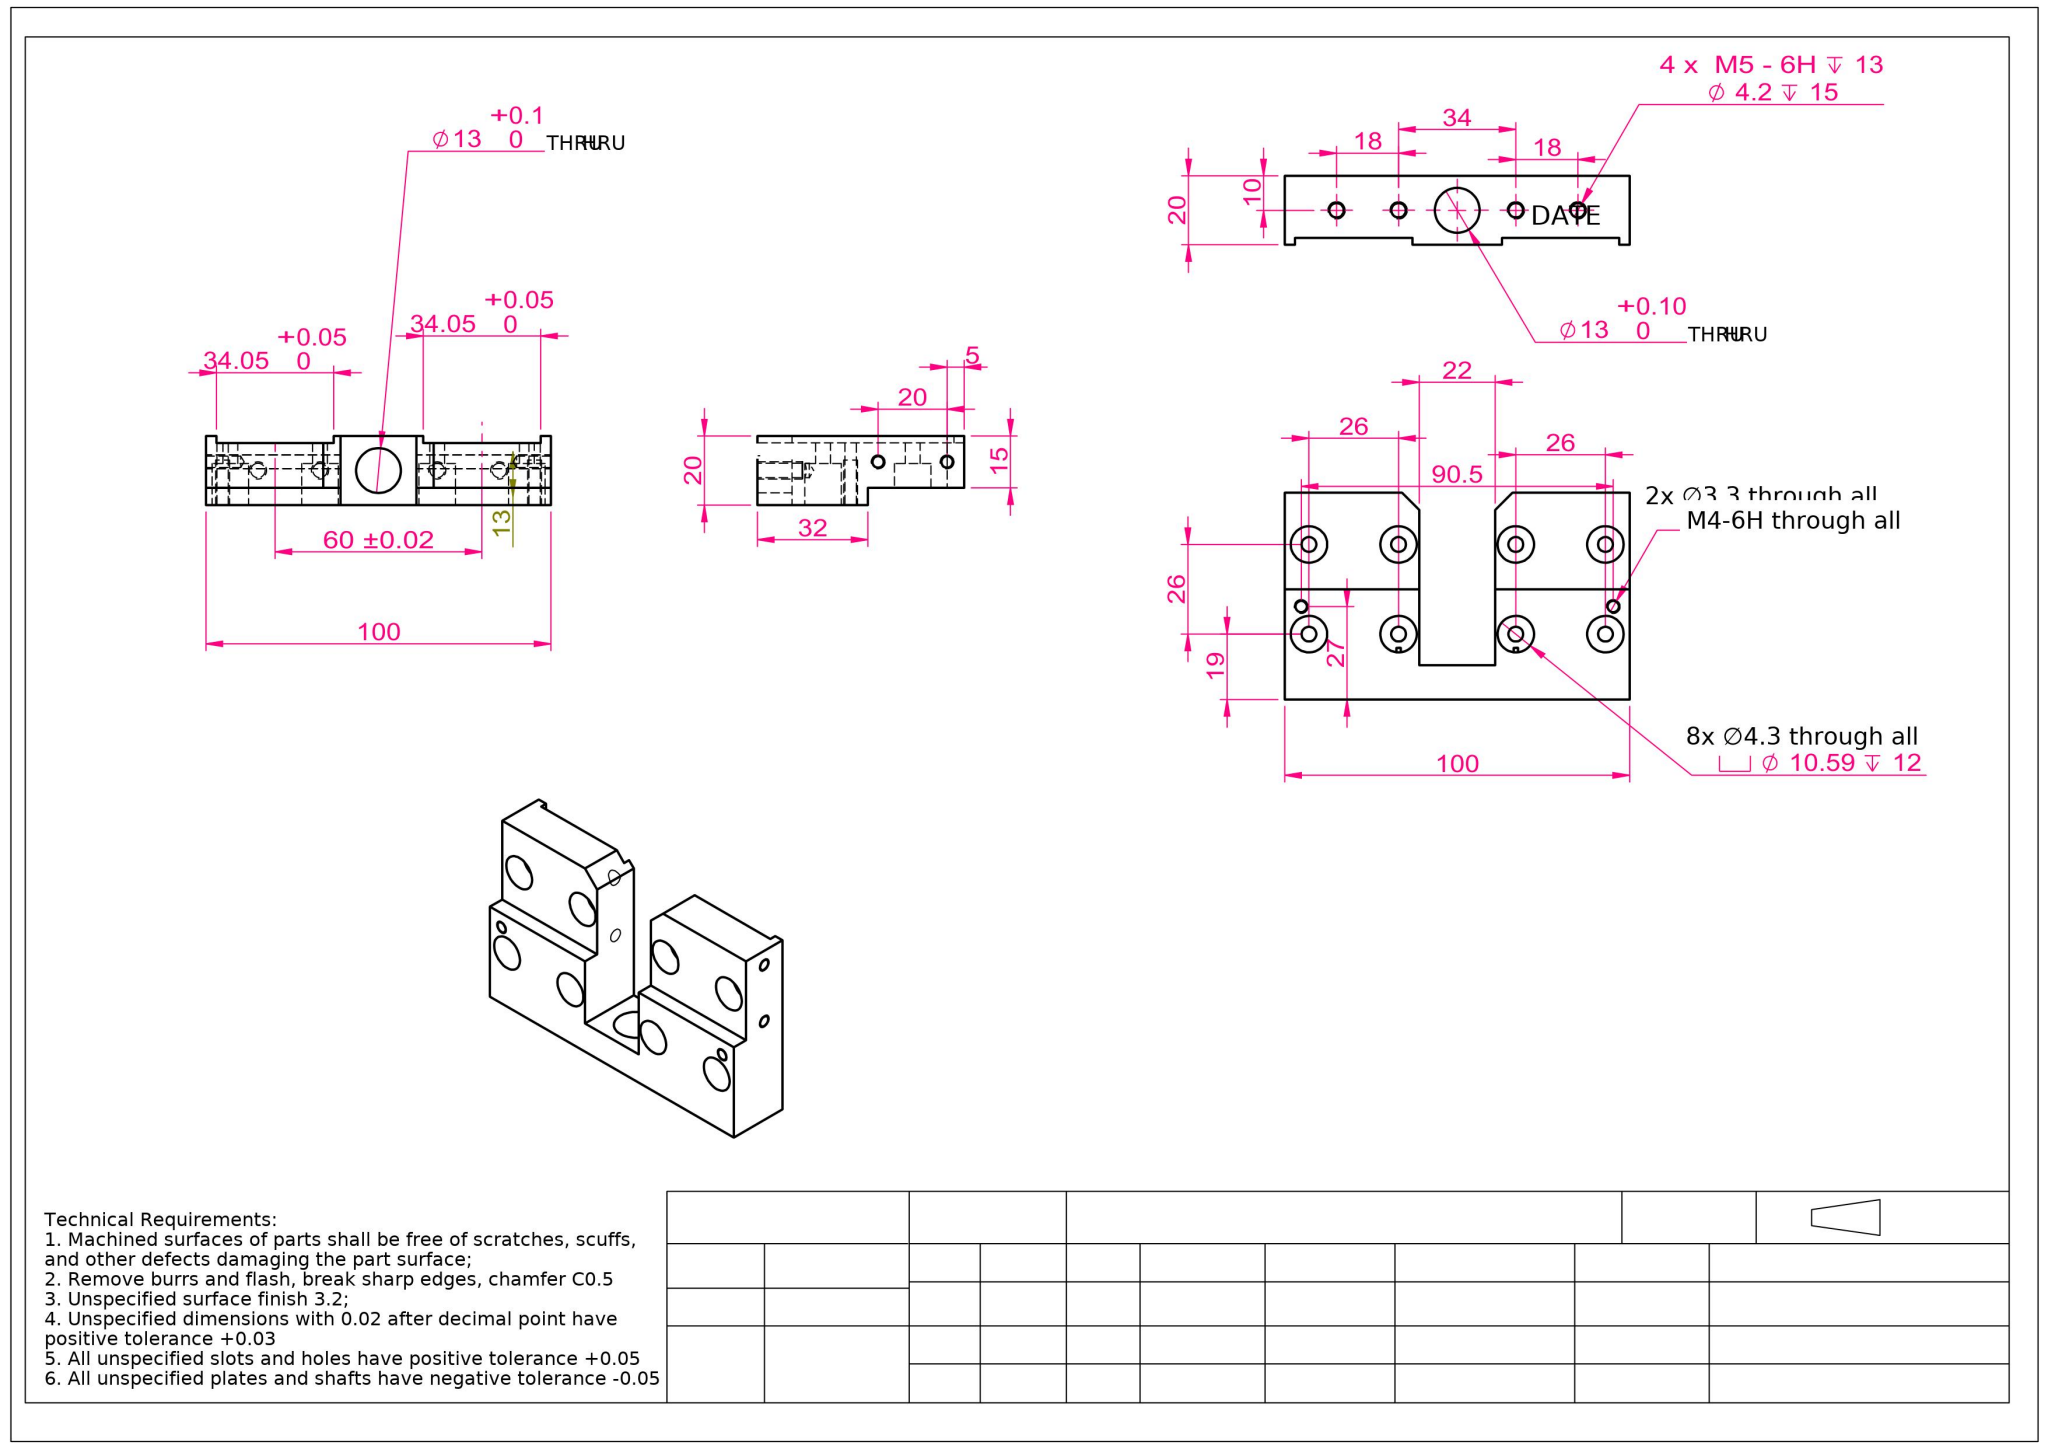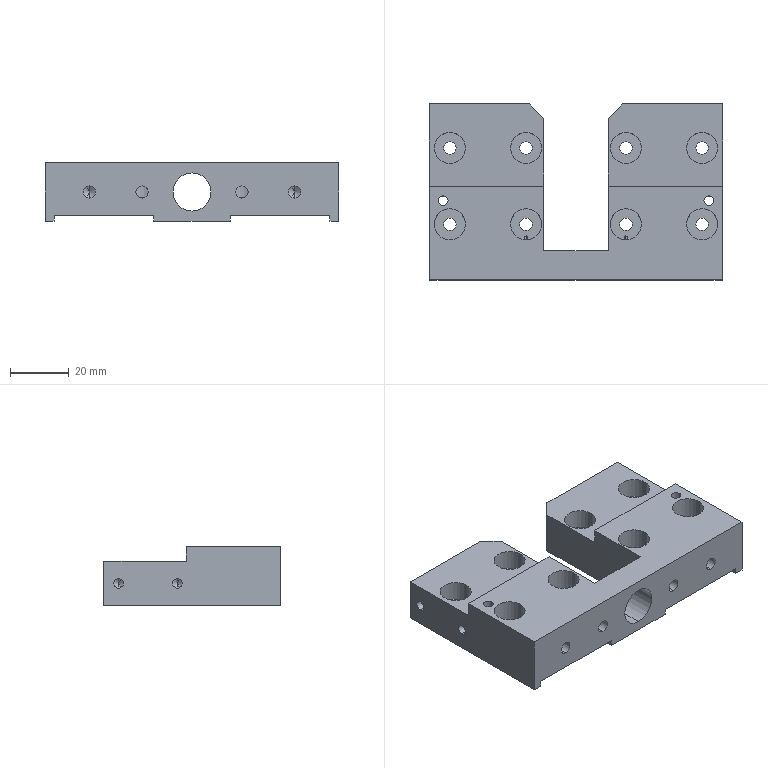Part | SolidWorks | mm | 1 solid | 102 faces | box 100 x 60 x 20 mm | volume 68361 mm3 | cylinder 54 | plane 32 | cone 16 | commonest cylinder face diameters 10.59 x16 4.3 x16 3.3 x12 4.2 x8 13 x2
build123d program:
from build123d import *

# Parameters (mm, degrees)
SKETCH1_W                                           = 100
SKETCH1_H                                           = 20
BOSS_EXTRUDE1_DEPTH                                 = 60
SKETCH3_W                                           = 34.05
SKETCH3_H                                           = 2
CUT_EXTRUDE2_DEPTH                                  = 79.74
CYLINDRICAL_COUNTERSUNK_HOLE_FOR_M4_HEX_D           = 4.3
CYLINDRICAL_COUNTERSUNK_HOLE_FOR_M4_HEX_CBORE_D     = 10.59
CYLINDRICAL_COUNTERSUNK_HOLE_FOR_M4_HEX_CBORE_DEPTH = 12
SKETCH9_R                                           = 6.5
CUT_EXTRUDE3_DEPTH                                  = 79.74
SKETCH10_W                                          = 22
SKETCH10_H                                          = 50
CUT_EXTRUDE4_DEPTH                                  = 65.226
M5_TAPPED_HOLE1_D                                   = 4.2
M5_TAPPED_HOLE1_DEPTH                               = 15
M5_TAPPED_HOLE1_TIP                                 = 1.262
M4_TAPPED_HOLE1_AT_2_COUNT                          = 2
M4_TAPPED_HOLE1_AT_2_PITCH                          = 20
M4_TAPPED_HOLE2_D                                   = 3.3
SKETCH19_W                                          = 100
SKETCH19_H                                          = 28
CUT_EXTRUDE5_DEPTH                                  = 5
CHAMFER2_SIZE                                       = 5


with BuildPart() as part:
    # Sketch1 → Boss-Extrude1 (new body)
    with BuildSketch(Plane(origin=(0, 25, 0), x_dir=(1, 0, 0), z_dir=(0, 1, 0))):
        Rectangle(SKETCH1_W, SKETCH1_H)
    extrude(amount=-BOSS_EXTRUDE1_DEPTH)

    # Sketch3 → Cut-Extrude2 (cut, through all)
    with BuildSketch(Plane.XZ.offset(35)):
        with Locations((-30, -9)):
            Rectangle(SKETCH3_W, SKETCH3_H)
        with Locations((30, -9)):
            Rectangle(SKETCH3_W, SKETCH3_H)
    extrude(amount=-CUT_EXTRUDE2_DEPTH, mode=Mode.SUBTRACT)

    # Cylindrical Countersunk Hole for M4 Hex (through all)
    with Locations(Plane.XY.offset(10)):
        with Locations((17, -16), (43, -16), (43, 10), (17, 10), (-43, 10), (-43, -16), (-17, 10), (-17, -16)):
            CounterBoreHole(CYLINDRICAL_COUNTERSUNK_HOLE_FOR_M4_HEX_D / 2, CYLINDRICAL_COUNTERSUNK_HOLE_FOR_M4_HEX_CBORE_D / 2, CYLINDRICAL_COUNTERSUNK_HOLE_FOR_M4_HEX_CBORE_DEPTH)

    # Sketch9 → Cut-Extrude3 (cut, through all)
    with BuildSketch(Plane(origin=(0, 25, 0), x_dir=(1, 0, 0), z_dir=(0, 1, 0))):
        with Locations(Location((0, 0, 0), (0, 0, 270))):
            Circle(SKETCH9_R)
    extrude(amount=-CUT_EXTRUDE3_DEPTH, mode=Mode.SUBTRACT)

    # Sketch10 → Cut-Extrude4 (cut, through all)
    with BuildSketch(Plane.XY.offset(10)):
        Rectangle(SKETCH10_W, SKETCH10_H)
    extrude(amount=-CUT_EXTRUDE4_DEPTH, mode=Mode.SUBTRACT)

    # M5 Tapped Hole1
    with Locations(Plane(origin=(0, -35, 0), x_dir=(-1, 0, 0), z_dir=(0, -1, 0))):
        with Locations((35, 0), (17, 0), (-17, 0), (-35, 0)):
            Hole(M5_TAPPED_HOLE1_D / 2, depth=M5_TAPPED_HOLE1_DEPTH)
            with Locations((0, 0, -(M5_TAPPED_HOLE1_DEPTH + M5_TAPPED_HOLE1_TIP / 2))):  # 118° drill point
                Cone(0, M5_TAPPED_HOLE1_D / 2, M5_TAPPED_HOLE1_TIP, mode=Mode.SUBTRACT)

    # Sketch16 → M4 Tapped Hole1 (revolve, cut)
    with BuildSketch(Plane(origin=(50, 20, -2.5), x_dir=(0, 0, -1), z_dir=(0, 1, 0))):
        Polygon((0, 0), (0, 10.991), (1.65, 10), (1.65, 0), align=None)
    m4_tapped_hole1 = revolve(axis=Axis((56.35, 20, -2.5), (-1, 0, 0)), mode=Mode.SUBTRACT)

    # M4 Tapped Hole1 at 2: M4 Tapped Hole1 ×2
    with Locations(*[(0, -i * M4_TAPPED_HOLE1_AT_2_PITCH, 0) for i in range(1, M4_TAPPED_HOLE1_AT_2_COUNT)]):
        add(m4_tapped_hole1, mode=Mode.SUBTRACT)

    # Mirror1: M4 Tapped Hole1 across plane
    add(m4_tapped_hole1.mirror(Plane(origin=(0, 0, 0), x_dir=(0, 0, 1), z_dir=(1, 0, 0))), mode=Mode.SUBTRACT)

    # Mirror1 copy 1 sketch → Mirror1 copy 1 (revolve, cut)
    with BuildSketch(Plane(origin=(-50, 0, -2.5), x_dir=(0, 0, -1), z_dir=(0, 1, 0))):
        Polygon((0, 0), (0, -10.991), (1.65, -10), (1.65, 0), align=None)
    revolve(axis=Axis((-56.35, 0, -2.5), (-1, 0, 0)), mode=Mode.SUBTRACT)

    # M4 Tapped Hole2 (through all)
    with Locations(Plane.XY.offset(10)):
        with Locations((-45.25, -8), (45.25, -8)):
            Hole(M4_TAPPED_HOLE2_D / 2)

    # Sketch19 → Cut-Extrude5 (cut)
    with BuildSketch(Plane.XY.offset(10)):
        with Locations((0, 11)):
            Rectangle(SKETCH19_W, SKETCH19_H)
    extrude(amount=-CUT_EXTRUDE5_DEPTH, mode=Mode.SUBTRACT)

    # Chamfer2
    chamfer2_edges = [part.edges().sort_by_distance(p)[0] for p in [
        (11, 25, -2.5),
        (-11, 25, -2.5),
    ]]
    chamfer(chamfer2_edges, length=CHAMFER2_SIZE)


solid = part.part